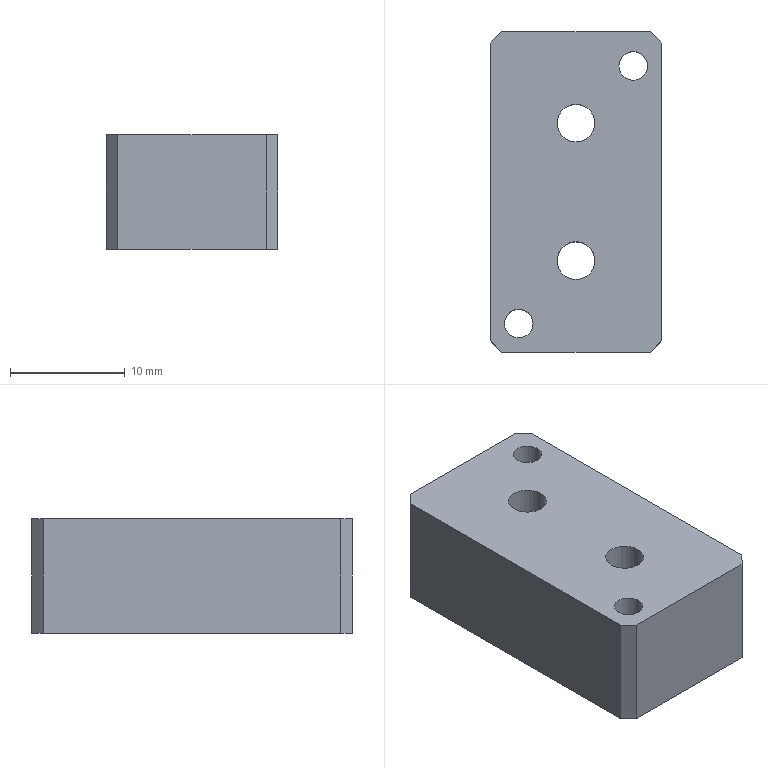Component | SolidWorks | JCT-03-04MicroSwitchMountingBlock-1 | 1 solid | 18 faces | box 15 x 28 x 10 mm | volume 3911 mm3 | plane 10 | cylinder 8 | commonest cylinder face diameters 2.5 x4 3.3 x4
build123d program:
from build123d import *

# Parameters (mm, degrees)
SKETCH1_W         = 15
SKETCH1_H         = 28
EXTRUDE1_DEPTH    = 5
M4_TAPPED_HOLE1_D = 3.3
M3_TAPPED_HOLE1_D = 2.5
CHAMFER1_SIZE     = 1


with BuildPart() as part:
    # Sketch1 → Extrude1 (new, symmetric)
    with BuildSketch(Plane.XY):
        Rectangle(SKETCH1_W, SKETCH1_H)
    extrude(amount=EXTRUDE1_DEPTH, both=True)

    # M4 Tapped Hole1 (through all)
    with Locations(Plane.XY.offset(5)):
        with Locations((0, -6), (0, 6)):
            Hole(M4_TAPPED_HOLE1_D / 2)

    # M3 Tapped Hole1 (through all)
    with Locations(Plane.XY.offset(5)):
        with Locations((5, 11), (-5, -11.5)):
            Hole(M3_TAPPED_HOLE1_D / 2)

    # Chamfer1
    chamfer1_edges = [part.edges().sort_by_distance(p)[0] for p in [
        (-7.5, 14, 0),
        (7.5, 14, 0),
        (7.5, -14, 0),
        (-7.5, -14, 0),
    ]]
    chamfer(chamfer1_edges, length=CHAMFER1_SIZE)


solid = part.part

# Placed as in the assembly
solid = solid.moved(Location((-12.734, 78.299, 51), (0, 0, 0)))
STEP:
#1=CARTESIAN_POINT('',(-0.3537,3.516,1.811));
#2=VERTEX_POINT('',#1);
#3=CARTESIAN_POINT('',(-0.2553,3.516,1.811));
#4=VERTEX_POINT('',#3);
#5=CARTESIAN_POINT('',(-0.3045,3.516,1.811));
#6=DIRECTION('',(0.,0.,1.));
#7=DIRECTION('',(1.,0.,0.));
#8=AXIS2_PLACEMENT_3D('',#5,#6,#7);
#9=CIRCLE('',#8,0.04921);
#10=EDGE_CURVE('',#2,#4,#9,.T.);
#11=ORIENTED_EDGE('',*,*,#10,.F.);
#12=CARTESIAN_POINT('',(-0.3537,3.516,2.205));
#13=VERTEX_POINT('',#12);
#14=CARTESIAN_POINT('',(-0.3537,3.516,2.205));
#15=DIRECTION('',(0.,0.,1.));
#16=VECTOR('',#15,39.37);
#17=LINE('',#14,#16);
#18=EDGE_CURVE('',#2,#13,#17,.T.);
#19=ORIENTED_EDGE('',*,*,#18,.T.);
#20=CARTESIAN_POINT('',(-0.2553,3.516,2.205));
#21=VERTEX_POINT('',#20);
#22=CARTESIAN_POINT('',(-0.3045,3.516,2.205));
#23=DIRECTION('',(0.,0.,1.));
#24=DIRECTION('',(1.,0.,0.));
#25=AXIS2_PLACEMENT_3D('',#22,#23,#24);
#26=CIRCLE('',#25,0.04921);
#27=EDGE_CURVE('',#13,#21,#26,.T.);
#28=ORIENTED_EDGE('',*,*,#27,.T.);
#29=CARTESIAN_POINT('',(-0.2553,3.516,2.205));
#30=DIRECTION('',(0.,0.,1.));
#31=VECTOR('',#30,39.37);
#32=LINE('',#29,#31);
#33=EDGE_CURVE('',#4,#21,#32,.T.);
#34=ORIENTED_EDGE('',*,*,#33,.F.);
#35=EDGE_LOOP('',(#11,#19,#28,#34));
#36=FACE_OUTER_BOUND('',#35,.T.);
#37=CARTESIAN_POINT('',(-0.3045,3.516,2.205));
#38=DIRECTION('',(0.,0.,1.));
#39=DIRECTION('',(1.,0.,0.));
#40=AXIS2_PLACEMENT_3D('',#37,#38,#39);
#41=CYLINDRICAL_SURFACE('',#40,0.04921);
#42=ADVANCED_FACE('',(#36),#41,.F.);
#43=CARTESIAN_POINT('',(-0.7474,2.63,1.811));
#44=VERTEX_POINT('',#43);
#45=CARTESIAN_POINT('',(-0.649,2.63,1.811));
#46=VERTEX_POINT('',#45);
#47=CARTESIAN_POINT('',(-0.6982,2.63,1.811));
#48=DIRECTION('',(0.,0.,1.));
#49=DIRECTION('',(1.,0.,0.));
#50=AXIS2_PLACEMENT_3D('',#47,#48,#49);
#51=CIRCLE('',#50,0.04921);
#52=EDGE_CURVE('',#44,#46,#51,.T.);
#53=ORIENTED_EDGE('',*,*,#52,.F.);
#54=CARTESIAN_POINT('',(-0.7474,2.63,2.205));
#55=VERTEX_POINT('',#54);
#56=CARTESIAN_POINT('',(-0.7474,2.63,2.205));
#57=DIRECTION('',(0.,0.,1.));
#58=VECTOR('',#57,39.37);
#59=LINE('',#56,#58);
#60=EDGE_CURVE('',#44,#55,#59,.T.);
#61=ORIENTED_EDGE('',*,*,#60,.T.);
#62=CARTESIAN_POINT('',(-0.649,2.63,2.205));
#63=VERTEX_POINT('',#62);
#64=CARTESIAN_POINT('',(-0.6982,2.63,2.205));
#65=DIRECTION('',(0.,0.,1.));
#66=DIRECTION('',(1.,0.,0.));
#67=AXIS2_PLACEMENT_3D('',#64,#65,#66);
#68=CIRCLE('',#67,0.04921);
#69=EDGE_CURVE('',#55,#63,#68,.T.);
#70=ORIENTED_EDGE('',*,*,#69,.T.);
#71=CARTESIAN_POINT('',(-0.649,2.63,2.205));
#72=DIRECTION('',(0.,0.,1.));
#73=VECTOR('',#72,39.37);
#74=LINE('',#71,#73);
#75=EDGE_CURVE('',#46,#63,#74,.T.);
#76=ORIENTED_EDGE('',*,*,#75,.F.);
#77=EDGE_LOOP('',(#53,#61,#70,#76));
#78=FACE_OUTER_BOUND('',#77,.T.);
#79=CARTESIAN_POINT('',(-0.6982,2.63,2.205));
#80=DIRECTION('',(0.,0.,1.));
#81=DIRECTION('',(1.,0.,0.));
#82=AXIS2_PLACEMENT_3D('',#79,#80,#81);
#83=CYLINDRICAL_SURFACE('',#82,0.04921);
#84=ADVANCED_FACE('',(#78),#83,.F.);
#85=CARTESIAN_POINT('',(-0.5663,3.319,1.811));
#86=VERTEX_POINT('',#85);
#87=CARTESIAN_POINT('',(-0.4364,3.319,1.811));
#88=VERTEX_POINT('',#87);
#89=CARTESIAN_POINT('',(-0.5013,3.319,1.811));
#90=DIRECTION('',(0.,0.,1.));
#91=DIRECTION('',(1.,0.,0.));
#92=AXIS2_PLACEMENT_3D('',#89,#90,#91);
#93=CIRCLE('',#92,0.06496);
#94=EDGE_CURVE('',#86,#88,#93,.T.);
#95=ORIENTED_EDGE('',*,*,#94,.F.);
#96=CARTESIAN_POINT('',(-0.5663,3.319,2.205));
#97=VERTEX_POINT('',#96);
#98=CARTESIAN_POINT('',(-0.5663,3.319,2.205));
#99=DIRECTION('',(0.,0.,1.));
#100=VECTOR('',#99,39.37);
#101=LINE('',#98,#100);
#102=EDGE_CURVE('',#86,#97,#101,.T.);
#103=ORIENTED_EDGE('',*,*,#102,.T.);
#104=CARTESIAN_POINT('',(-0.4364,3.319,2.205));
#105=VERTEX_POINT('',#104);
#106=CARTESIAN_POINT('',(-0.5013,3.319,2.205));
#107=DIRECTION('',(0.,0.,1.));
#108=DIRECTION('',(1.,0.,0.));
#109=AXIS2_PLACEMENT_3D('',#106,#107,#108);
#110=CIRCLE('',#109,0.06496);
#111=EDGE_CURVE('',#97,#105,#110,.T.);
#112=ORIENTED_EDGE('',*,*,#111,.T.);
#113=CARTESIAN_POINT('',(-0.4364,3.319,2.205));
#114=DIRECTION('',(0.,0.,1.));
#115=VECTOR('',#114,39.37);
#116=LINE('',#113,#115);
#117=EDGE_CURVE('',#88,#105,#116,.T.);
#118=ORIENTED_EDGE('',*,*,#117,.F.);
#119=EDGE_LOOP('',(#95,#103,#112,#118));
#120=FACE_OUTER_BOUND('',#119,.T.);
#121=CARTESIAN_POINT('',(-0.5013,3.319,2.205));
#122=DIRECTION('',(0.,0.,1.));
#123=DIRECTION('',(1.,0.,0.));
#124=AXIS2_PLACEMENT_3D('',#121,#122,#123);
#125=CYLINDRICAL_SURFACE('',#124,0.06496);
#126=ADVANCED_FACE('',(#120),#125,.F.);
#127=CARTESIAN_POINT('',(-0.5663,2.846,1.811));
#128=VERTEX_POINT('',#127);
#129=CARTESIAN_POINT('',(-0.4364,2.846,1.811));
#130=VERTEX_POINT('',#129);
#131=CARTESIAN_POINT('',(-0.5013,2.846,1.811));
#132=DIRECTION('',(0.,0.,1.));
#133=DIRECTION('',(1.,0.,0.));
#134=AXIS2_PLACEMENT_3D('',#131,#132,#133);
#135=CIRCLE('',#134,0.06496);
#136=EDGE_CURVE('',#128,#130,#135,.T.);
#137=ORIENTED_EDGE('',*,*,#136,.F.);
#138=CARTESIAN_POINT('',(-0.5663,2.846,2.205));
#139=VERTEX_POINT('',#138);
#140=CARTESIAN_POINT('',(-0.5663,2.846,2.205));
#141=DIRECTION('',(0.,0.,1.));
#142=VECTOR('',#141,39.37);
#143=LINE('',#140,#142);
#144=EDGE_CURVE('',#128,#139,#143,.T.);
#145=ORIENTED_EDGE('',*,*,#144,.T.);
#146=CARTESIAN_POINT('',(-0.4364,2.846,2.205));
#147=VERTEX_POINT('',#146);
#148=CARTESIAN_POINT('',(-0.5013,2.846,2.205));
#149=DIRECTION('',(0.,0.,1.));
#150=DIRECTION('',(1.,0.,0.));
#151=AXIS2_PLACEMENT_3D('',#148,#149,#150);
#152=CIRCLE('',#151,0.06496);
#153=EDGE_CURVE('',#139,#147,#152,.T.);
#154=ORIENTED_EDGE('',*,*,#153,.T.);
#155=CARTESIAN_POINT('',(-0.4364,2.846,2.205));
#156=DIRECTION('',(0.,0.,1.));
#157=VECTOR('',#156,39.37);
#158=LINE('',#155,#157);
#159=EDGE_CURVE('',#130,#147,#158,.T.);
#160=ORIENTED_EDGE('',*,*,#159,.F.);
#161=EDGE_LOOP('',(#137,#145,#154,#160));
#162=FACE_OUTER_BOUND('',#161,.T.);
#163=CARTESIAN_POINT('',(-0.5013,2.846,2.205));
#164=DIRECTION('',(0.,0.,1.));
#165=DIRECTION('',(1.,0.,0.));
#166=AXIS2_PLACEMENT_3D('',#163,#164,#165);
#167=CYLINDRICAL_SURFACE('',#166,0.06496);
#168=ADVANCED_FACE('',(#162),#167,.F.);
#169=CARTESIAN_POINT('',(-0.7966,3.594,1.811));
#170=VERTEX_POINT('',#169);
#171=CARTESIAN_POINT('',(-0.7966,2.571,1.811));
#172=VERTEX_POINT('',#171);
#173=CARTESIAN_POINT('',(-0.7966,3.634,1.811));
#174=DIRECTION('',(0.,-1.,0.));
#175=VECTOR('',#174,39.37);
#176=LINE('',#173,#175);
#177=EDGE_CURVE('',#170,#172,#176,.T.);
#178=ORIENTED_EDGE('',*,*,#177,.T.);
#179=CARTESIAN_POINT('',(-0.7966,2.571,2.205));
#180=VERTEX_POINT('',#179);
#181=CARTESIAN_POINT('',(-0.7966,2.571,2.205));
#182=DIRECTION('',(0.,0.,1.));
#183=VECTOR('',#182,39.37);
#184=LINE('',#181,#183);
#185=EDGE_CURVE('',#172,#180,#184,.T.);
#186=ORIENTED_EDGE('',*,*,#185,.T.);
#187=CARTESIAN_POINT('',(-0.7966,3.594,2.205));
#188=VERTEX_POINT('',#187);
#189=CARTESIAN_POINT('',(-0.7966,3.634,2.205));
#190=DIRECTION('',(0.,-1.,0.));
#191=VECTOR('',#190,39.37);
#192=LINE('',#189,#191);
#193=EDGE_CURVE('',#188,#180,#192,.T.);
#194=ORIENTED_EDGE('',*,*,#193,.F.);
#195=CARTESIAN_POINT('',(-0.7966,3.594,2.205));
#196=DIRECTION('',(0.,0.,-1.));
#197=VECTOR('',#196,39.37);
#198=LINE('',#195,#197);
#199=EDGE_CURVE('',#188,#170,#198,.T.);
#200=ORIENTED_EDGE('',*,*,#199,.T.);
#201=EDGE_LOOP('',(#178,#186,#194,#200));
#202=FACE_OUTER_BOUND('',#201,.T.);
#203=CARTESIAN_POINT('',(-0.7966,3.634,2.205));
#204=DIRECTION('',(1.,0.,0.));
#205=DIRECTION('',(0.,0.,-1.));
#206=AXIS2_PLACEMENT_3D('',#203,#204,#205);
#207=PLANE('',#206);
#208=ADVANCED_FACE('',(#202),#207,.F.);
#209=CARTESIAN_POINT('',(-0.7572,2.531,2.205));
#210=VERTEX_POINT('',#209);
#211=CARTESIAN_POINT('',(-0.2454,2.531,2.205));
#212=VERTEX_POINT('',#211);
#213=CARTESIAN_POINT('',(-0.7966,2.531,2.205));
#214=DIRECTION('',(1.,-0.,0.));
#215=VECTOR('',#214,39.37);
#216=LINE('',#213,#215);
#217=EDGE_CURVE('',#210,#212,#216,.T.);
#218=ORIENTED_EDGE('',*,*,#217,.F.);
#219=CARTESIAN_POINT('',(-0.7572,2.531,1.811));
#220=VERTEX_POINT('',#219);
#221=CARTESIAN_POINT('',(-0.7572,2.531,2.205));
#222=DIRECTION('',(0.,0.,-1.));
#223=VECTOR('',#222,39.37);
#224=LINE('',#221,#223);
#225=EDGE_CURVE('',#210,#220,#224,.T.);
#226=ORIENTED_EDGE('',*,*,#225,.T.);
#227=CARTESIAN_POINT('',(-0.2454,2.531,1.811));
#228=VERTEX_POINT('',#227);
#229=CARTESIAN_POINT('',(-0.7966,2.531,1.811));
#230=DIRECTION('',(1.,-0.,0.));
#231=VECTOR('',#230,39.37);
#232=LINE('',#229,#231);
#233=EDGE_CURVE('',#220,#228,#232,.T.);
#234=ORIENTED_EDGE('',*,*,#233,.T.);
#235=CARTESIAN_POINT('',(-0.2454,2.531,2.205));
#236=DIRECTION('',(0.,0.,1.));
#237=VECTOR('',#236,39.37);
#238=LINE('',#235,#237);
#239=EDGE_CURVE('',#228,#212,#238,.T.);
#240=ORIENTED_EDGE('',*,*,#239,.T.);
#241=EDGE_LOOP('',(#218,#226,#234,#240));
#242=FACE_OUTER_BOUND('',#241,.T.);
#243=CARTESIAN_POINT('',(-0.7966,2.531,2.205));
#244=DIRECTION('',(0.,1.,0.));
#245=DIRECTION('',(-1.,0.,0.));
#246=AXIS2_PLACEMENT_3D('',#243,#244,#245);
#247=PLANE('',#246);
#248=ADVANCED_FACE('',(#242),#247,.F.);
#249=CARTESIAN_POINT('',(-0.2061,2.571,2.205));
#250=VERTEX_POINT('',#249);
#251=CARTESIAN_POINT('',(-0.2061,3.594,2.205));
#252=VERTEX_POINT('',#251);
#253=CARTESIAN_POINT('',(-0.2061,3.634,2.205));
#254=DIRECTION('',(0.,1.,0.));
#255=VECTOR('',#254,39.37);
#256=LINE('',#253,#255);
#257=EDGE_CURVE('',#250,#252,#256,.T.);
#258=ORIENTED_EDGE('',*,*,#257,.F.);
#259=CARTESIAN_POINT('',(-0.2061,2.571,1.811));
#260=VERTEX_POINT('',#259);
#261=CARTESIAN_POINT('',(-0.2061,2.571,2.205));
#262=DIRECTION('',(0.,0.,-1.));
#263=VECTOR('',#262,39.37);
#264=LINE('',#261,#263);
#265=EDGE_CURVE('',#250,#260,#264,.T.);
#266=ORIENTED_EDGE('',*,*,#265,.T.);
#267=CARTESIAN_POINT('',(-0.2061,3.594,1.811));
#268=VERTEX_POINT('',#267);
#269=CARTESIAN_POINT('',(-0.2061,3.634,1.811));
#270=DIRECTION('',(0.,1.,0.));
#271=VECTOR('',#270,39.37);
#272=LINE('',#269,#271);
#273=EDGE_CURVE('',#260,#268,#272,.T.);
#274=ORIENTED_EDGE('',*,*,#273,.T.);
#275=CARTESIAN_POINT('',(-0.2061,3.594,2.205));
#276=DIRECTION('',(0.,0.,1.));
#277=VECTOR('',#276,39.37);
#278=LINE('',#275,#277);
#279=EDGE_CURVE('',#268,#252,#278,.T.);
#280=ORIENTED_EDGE('',*,*,#279,.T.);
#281=EDGE_LOOP('',(#258,#266,#274,#280));
#282=FACE_OUTER_BOUND('',#281,.T.);
#283=CARTESIAN_POINT('',(-0.2061,3.634,2.205));
#284=DIRECTION('',(-1.,0.,0.));
#285=DIRECTION('',(0.,0.,1.));
#286=AXIS2_PLACEMENT_3D('',#283,#284,#285);
#287=PLANE('',#286);
#288=ADVANCED_FACE('',(#282),#287,.F.);
#289=CARTESIAN_POINT('',(-0.2454,3.634,2.205));
#290=VERTEX_POINT('',#289);
#291=CARTESIAN_POINT('',(-0.7572,3.634,2.205));
#292=VERTEX_POINT('',#291);
#293=CARTESIAN_POINT('',(-0.7966,3.634,2.205));
#294=DIRECTION('',(-1.,0.,0.));
#295=VECTOR('',#294,39.37);
#296=LINE('',#293,#295);
#297=EDGE_CURVE('',#290,#292,#296,.T.);
#298=ORIENTED_EDGE('',*,*,#297,.F.);
#299=CARTESIAN_POINT('',(-0.2454,3.634,1.811));
#300=VERTEX_POINT('',#299);
#301=CARTESIAN_POINT('',(-0.2454,3.634,2.205));
#302=DIRECTION('',(0.,0.,-1.));
#303=VECTOR('',#302,39.37);
#304=LINE('',#301,#303);
#305=EDGE_CURVE('',#290,#300,#304,.T.);
#306=ORIENTED_EDGE('',*,*,#305,.T.);
#307=CARTESIAN_POINT('',(-0.7572,3.634,1.811));
#308=VERTEX_POINT('',#307);
#309=CARTESIAN_POINT('',(-0.7966,3.634,1.811));
#310=DIRECTION('',(-1.,0.,0.));
#311=VECTOR('',#310,39.37);
#312=LINE('',#309,#311);
#313=EDGE_CURVE('',#300,#308,#312,.T.);
#314=ORIENTED_EDGE('',*,*,#313,.T.);
#315=CARTESIAN_POINT('',(-0.7572,3.634,2.205));
#316=DIRECTION('',(0.,0.,1.));
#317=VECTOR('',#316,39.37);
#318=LINE('',#315,#317);
#319=EDGE_CURVE('',#308,#292,#318,.T.);
#320=ORIENTED_EDGE('',*,*,#319,.T.);
#321=EDGE_LOOP('',(#298,#306,#314,#320));
#322=FACE_OUTER_BOUND('',#321,.T.);
#323=CARTESIAN_POINT('',(-0.7966,3.634,2.205));
#324=DIRECTION('',(0.,-1.,0.));
#325=DIRECTION('',(0.,0.,-1.));
#326=AXIS2_PLACEMENT_3D('',#323,#324,#325);
#327=PLANE('',#326);
#328=ADVANCED_FACE('',(#322),#327,.F.);
#329=CARTESIAN_POINT('',(-0.3045,3.516,2.205));
#330=DIRECTION('',(0.,0.,1.));
#331=DIRECTION('',(1.,0.,0.));
#332=AXIS2_PLACEMENT_3D('',#329,#330,#331);
#333=CIRCLE('',#332,0.04921);
#334=EDGE_CURVE('',#21,#13,#333,.T.);
#335=ORIENTED_EDGE('',*,*,#334,.F.);
#336=ORIENTED_EDGE('',*,*,#27,.F.);
#337=EDGE_LOOP('',(#335,#336));
#338=FACE_BOUND('',#337,.T.);
#339=CARTESIAN_POINT('',(-0.6982,2.63,2.205));
#340=DIRECTION('',(0.,0.,1.));
#341=DIRECTION('',(1.,0.,0.));
#342=AXIS2_PLACEMENT_3D('',#339,#340,#341);
#343=CIRCLE('',#342,0.04921);
#344=EDGE_CURVE('',#63,#55,#343,.T.);
#345=ORIENTED_EDGE('',*,*,#344,.F.);
#346=ORIENTED_EDGE('',*,*,#69,.F.);
#347=EDGE_LOOP('',(#345,#346));
#348=FACE_BOUND('',#347,.T.);
#349=CARTESIAN_POINT('',(-0.5013,3.319,2.205));
#350=DIRECTION('',(0.,0.,1.));
#351=DIRECTION('',(1.,0.,0.));
#352=AXIS2_PLACEMENT_3D('',#349,#350,#351);
#353=CIRCLE('',#352,0.06496);
#354=EDGE_CURVE('',#105,#97,#353,.T.);
#355=ORIENTED_EDGE('',*,*,#354,.F.);
#356=ORIENTED_EDGE('',*,*,#111,.F.);
#357=EDGE_LOOP('',(#355,#356));
#358=FACE_BOUND('',#357,.T.);
#359=CARTESIAN_POINT('',(-0.5013,2.846,2.205));
#360=DIRECTION('',(0.,0.,1.));
#361=DIRECTION('',(1.,0.,0.));
#362=AXIS2_PLACEMENT_3D('',#359,#360,#361);
#363=CIRCLE('',#362,0.06496);
#364=EDGE_CURVE('',#147,#139,#363,.T.);
#365=ORIENTED_EDGE('',*,*,#364,.F.);
#366=ORIENTED_EDGE('',*,*,#153,.F.);
#367=EDGE_LOOP('',(#365,#366));
#368=FACE_BOUND('',#367,.T.);
#369=ORIENTED_EDGE('',*,*,#193,.T.);
#370=CARTESIAN_POINT('',(-0.7769,2.551,2.205));
#371=DIRECTION('',(0.7071,-0.7071,0.));
#372=VECTOR('',#371,39.37);
#373=LINE('',#370,#372);
#374=EDGE_CURVE('',#180,#210,#373,.T.);
#375=ORIENTED_EDGE('',*,*,#374,.T.);
#376=ORIENTED_EDGE('',*,*,#217,.T.);
#377=CARTESIAN_POINT('',(-0.521,2.256,2.205));
#378=DIRECTION('',(0.7071,0.7071,0.));
#379=VECTOR('',#378,39.37);
#380=LINE('',#377,#379);
#381=EDGE_CURVE('',#212,#250,#380,.T.);
#382=ORIENTED_EDGE('',*,*,#381,.T.);
#383=ORIENTED_EDGE('',*,*,#257,.T.);
#384=CARTESIAN_POINT('',(0.03017,3.358,2.205));
#385=DIRECTION('',(-0.7071,0.7071,0.));
#386=VECTOR('',#385,39.37);
#387=LINE('',#384,#386);
#388=EDGE_CURVE('',#252,#290,#387,.T.);
#389=ORIENTED_EDGE('',*,*,#388,.T.);
#390=ORIENTED_EDGE('',*,*,#297,.T.);
#391=CARTESIAN_POINT('',(-1.328,3.063,2.205));
#392=DIRECTION('',(-0.7071,-0.7071,0.));
#393=VECTOR('',#392,39.37);
#394=LINE('',#391,#393);
#395=EDGE_CURVE('',#292,#188,#394,.T.);
#396=ORIENTED_EDGE('',*,*,#395,.T.);
#397=EDGE_LOOP('',(#369,#375,#376,#382,#383,#389,#390,#396));
#398=FACE_OUTER_BOUND('',#397,.T.);
#399=CARTESIAN_POINT('',(-0.7966,2.531,2.205));
#400=DIRECTION('',(0.,0.,1.));
#401=DIRECTION('',(1.,0.,0.));
#402=AXIS2_PLACEMENT_3D('',#399,#400,#401);
#403=PLANE('',#402);
#404=ADVANCED_FACE('',(#338,#348,#358,#368,#398),#403,.T.);
#405=CARTESIAN_POINT('',(-0.3045,3.516,1.811));
#406=DIRECTION('',(0.,0.,1.));
#407=DIRECTION('',(1.,0.,0.));
#408=AXIS2_PLACEMENT_3D('',#405,#406,#407);
#409=CIRCLE('',#408,0.04921);
#410=EDGE_CURVE('',#4,#2,#409,.T.);
#411=ORIENTED_EDGE('',*,*,#410,.T.);
#412=ORIENTED_EDGE('',*,*,#10,.T.);
#413=EDGE_LOOP('',(#411,#412));
#414=FACE_BOUND('',#413,.T.);
#415=CARTESIAN_POINT('',(-0.6982,2.63,1.811));
#416=DIRECTION('',(0.,0.,1.));
#417=DIRECTION('',(1.,0.,0.));
#418=AXIS2_PLACEMENT_3D('',#415,#416,#417);
#419=CIRCLE('',#418,0.04921);
#420=EDGE_CURVE('',#46,#44,#419,.T.);
#421=ORIENTED_EDGE('',*,*,#420,.T.);
#422=ORIENTED_EDGE('',*,*,#52,.T.);
#423=EDGE_LOOP('',(#421,#422));
#424=FACE_BOUND('',#423,.T.);
#425=CARTESIAN_POINT('',(-0.5013,3.319,1.811));
#426=DIRECTION('',(0.,0.,1.));
#427=DIRECTION('',(1.,0.,0.));
#428=AXIS2_PLACEMENT_3D('',#425,#426,#427);
#429=CIRCLE('',#428,0.06496);
#430=EDGE_CURVE('',#88,#86,#429,.T.);
#431=ORIENTED_EDGE('',*,*,#430,.T.);
#432=ORIENTED_EDGE('',*,*,#94,.T.);
#433=EDGE_LOOP('',(#431,#432));
#434=FACE_BOUND('',#433,.T.);
#435=CARTESIAN_POINT('',(-0.5013,2.846,1.811));
#436=DIRECTION('',(0.,0.,1.));
#437=DIRECTION('',(1.,0.,0.));
#438=AXIS2_PLACEMENT_3D('',#435,#436,#437);
#439=CIRCLE('',#438,0.06496);
#440=EDGE_CURVE('',#130,#128,#439,.T.);
#441=ORIENTED_EDGE('',*,*,#440,.T.);
#442=ORIENTED_EDGE('',*,*,#136,.T.);
#443=EDGE_LOOP('',(#441,#442));
#444=FACE_BOUND('',#443,.T.);
#445=ORIENTED_EDGE('',*,*,#233,.F.);
#446=CARTESIAN_POINT('',(-0.7572,2.531,1.811));
#447=DIRECTION('',(-0.7071,0.7071,0.));
#448=VECTOR('',#447,39.37);
#449=LINE('',#446,#448);
#450=EDGE_CURVE('',#220,#172,#449,.T.);
#451=ORIENTED_EDGE('',*,*,#450,.T.);
#452=ORIENTED_EDGE('',*,*,#177,.F.);
#453=CARTESIAN_POINT('',(-0.7966,3.594,1.811));
#454=DIRECTION('',(0.7071,0.7071,0.));
#455=VECTOR('',#454,39.37);
#456=LINE('',#453,#455);
#457=EDGE_CURVE('',#170,#308,#456,.T.);
#458=ORIENTED_EDGE('',*,*,#457,.T.);
#459=ORIENTED_EDGE('',*,*,#313,.F.);
#460=CARTESIAN_POINT('',(-0.2454,3.634,1.811));
#461=DIRECTION('',(0.7071,-0.7071,0.));
#462=VECTOR('',#461,39.37);
#463=LINE('',#460,#462);
#464=EDGE_CURVE('',#300,#268,#463,.T.);
#465=ORIENTED_EDGE('',*,*,#464,.T.);
#466=ORIENTED_EDGE('',*,*,#273,.F.);
#467=CARTESIAN_POINT('',(-0.2061,2.571,1.811));
#468=DIRECTION('',(-0.7071,-0.7071,0.));
#469=VECTOR('',#468,39.37);
#470=LINE('',#467,#469);
#471=EDGE_CURVE('',#260,#228,#470,.T.);
#472=ORIENTED_EDGE('',*,*,#471,.T.);
#473=EDGE_LOOP('',(#445,#451,#452,#458,#459,#465,#466,#472));
#474=FACE_OUTER_BOUND('',#473,.T.);
#475=CARTESIAN_POINT('',(-0.7966,2.531,1.811));
#476=DIRECTION('',(0.,0.,1.));
#477=DIRECTION('',(1.,0.,0.));
#478=AXIS2_PLACEMENT_3D('',#475,#476,#477);
#479=PLANE('',#478);
#480=ADVANCED_FACE('',(#414,#424,#434,#444,#474),#479,.F.);
#481=ORIENTED_EDGE('',*,*,#144,.F.);
#482=ORIENTED_EDGE('',*,*,#440,.F.);
#483=ORIENTED_EDGE('',*,*,#159,.T.);
#484=ORIENTED_EDGE('',*,*,#364,.T.);
#485=EDGE_LOOP('',(#481,#482,#483,#484));
#486=FACE_OUTER_BOUND('',#485,.T.);
#487=CARTESIAN_POINT('',(-0.5013,2.846,2.205));
#488=DIRECTION('',(0.,0.,1.));
#489=DIRECTION('',(1.,0.,0.));
#490=AXIS2_PLACEMENT_3D('',#487,#488,#489);
#491=CYLINDRICAL_SURFACE('',#490,0.06496);
#492=ADVANCED_FACE('',(#486),#491,.F.);
#493=ORIENTED_EDGE('',*,*,#102,.F.);
#494=ORIENTED_EDGE('',*,*,#430,.F.);
#495=ORIENTED_EDGE('',*,*,#117,.T.);
#496=ORIENTED_EDGE('',*,*,#354,.T.);
#497=EDGE_LOOP('',(#493,#494,#495,#496));
#498=FACE_OUTER_BOUND('',#497,.T.);
#499=CARTESIAN_POINT('',(-0.5013,3.319,2.205));
#500=DIRECTION('',(0.,0.,1.));
#501=DIRECTION('',(1.,0.,0.));
#502=AXIS2_PLACEMENT_3D('',#499,#500,#501);
#503=CYLINDRICAL_SURFACE('',#502,0.06496);
#504=ADVANCED_FACE('',(#498),#503,.F.);
#505=ORIENTED_EDGE('',*,*,#60,.F.);
#506=ORIENTED_EDGE('',*,*,#420,.F.);
#507=ORIENTED_EDGE('',*,*,#75,.T.);
#508=ORIENTED_EDGE('',*,*,#344,.T.);
#509=EDGE_LOOP('',(#505,#506,#507,#508));
#510=FACE_OUTER_BOUND('',#509,.T.);
#511=CARTESIAN_POINT('',(-0.6982,2.63,2.205));
#512=DIRECTION('',(0.,0.,1.));
#513=DIRECTION('',(1.,0.,0.));
#514=AXIS2_PLACEMENT_3D('',#511,#512,#513);
#515=CYLINDRICAL_SURFACE('',#514,0.04921);
#516=ADVANCED_FACE('',(#510),#515,.F.);
#517=ORIENTED_EDGE('',*,*,#18,.F.);
#518=ORIENTED_EDGE('',*,*,#410,.F.);
#519=ORIENTED_EDGE('',*,*,#33,.T.);
#520=ORIENTED_EDGE('',*,*,#334,.T.);
#521=EDGE_LOOP('',(#517,#518,#519,#520));
#522=FACE_OUTER_BOUND('',#521,.T.);
#523=CARTESIAN_POINT('',(-0.3045,3.516,2.205));
#524=DIRECTION('',(0.,0.,1.));
#525=DIRECTION('',(1.,0.,0.));
#526=AXIS2_PLACEMENT_3D('',#523,#524,#525);
#527=CYLINDRICAL_SURFACE('',#526,0.04921);
#528=ADVANCED_FACE('',(#522),#527,.F.);
#529=ORIENTED_EDGE('',*,*,#374,.F.);
#530=ORIENTED_EDGE('',*,*,#185,.F.);
#531=ORIENTED_EDGE('',*,*,#450,.F.);
#532=ORIENTED_EDGE('',*,*,#225,.F.);
#533=EDGE_LOOP('',(#529,#530,#531,#532));
#534=FACE_OUTER_BOUND('',#533,.T.);
#535=CARTESIAN_POINT('',(-0.7572,2.531,2.205));
#536=DIRECTION('',(0.7071,0.7071,0.));
#537=DIRECTION('',(-0.7071,0.7071,0.));
#538=AXIS2_PLACEMENT_3D('',#535,#536,#537);
#539=PLANE('',#538);
#540=ADVANCED_FACE('',(#534),#539,.F.);
#541=ORIENTED_EDGE('',*,*,#381,.F.);
#542=ORIENTED_EDGE('',*,*,#239,.F.);
#543=ORIENTED_EDGE('',*,*,#471,.F.);
#544=ORIENTED_EDGE('',*,*,#265,.F.);
#545=EDGE_LOOP('',(#541,#542,#543,#544));
#546=FACE_OUTER_BOUND('',#545,.T.);
#547=CARTESIAN_POINT('',(-0.2061,2.571,2.205));
#548=DIRECTION('',(-0.7071,0.7071,0.));
#549=DIRECTION('',(-0.7071,-0.7071,0.));
#550=AXIS2_PLACEMENT_3D('',#547,#548,#549);
#551=PLANE('',#550);
#552=ADVANCED_FACE('',(#546),#551,.F.);
#553=ORIENTED_EDGE('',*,*,#388,.F.);
#554=ORIENTED_EDGE('',*,*,#279,.F.);
#555=ORIENTED_EDGE('',*,*,#464,.F.);
#556=ORIENTED_EDGE('',*,*,#305,.F.);
#557=EDGE_LOOP('',(#553,#554,#555,#556));
#558=FACE_OUTER_BOUND('',#557,.T.);
#559=CARTESIAN_POINT('',(-0.2454,3.634,2.205));
#560=DIRECTION('',(-0.7071,-0.7071,0.));
#561=DIRECTION('',(0.7071,-0.7071,0.));
#562=AXIS2_PLACEMENT_3D('',#559,#560,#561);
#563=PLANE('',#562);
#564=ADVANCED_FACE('',(#558),#563,.F.);
#565=ORIENTED_EDGE('',*,*,#395,.F.);
#566=ORIENTED_EDGE('',*,*,#319,.F.);
#567=ORIENTED_EDGE('',*,*,#457,.F.);
#568=ORIENTED_EDGE('',*,*,#199,.F.);
#569=EDGE_LOOP('',(#565,#566,#567,#568));
#570=FACE_OUTER_BOUND('',#569,.T.);
#571=CARTESIAN_POINT('',(-0.7966,3.594,2.205));
#572=DIRECTION('',(0.7071,-0.7071,0.));
#573=DIRECTION('',(0.7071,0.7071,0.));
#574=AXIS2_PLACEMENT_3D('',#571,#572,#573);
#575=PLANE('',#574);
#576=ADVANCED_FACE('',(#570),#575,.F.);
#577=CLOSED_SHELL('',(#42,#84,#126,#168,#208,#248,#288,#328,#404,#480,#492,#504,#516,#528,#540,#552,#564,#576));
#578=MANIFOLD_SOLID_BREP('',#577);
#579=CARTESIAN_POINT('',(0.,0.,0.));
#580=DIRECTION('',(0.,0.,1.));
#581=DIRECTION('',(1.,0.,0.));
#582=AXIS2_PLACEMENT_3D('',#579,#580,#581);
#583=(LENGTH_UNIT()NAMED_UNIT(*)SI_UNIT($,.METRE.));
#584=LENGTH_MEASURE_WITH_UNIT(LENGTH_MEASURE(0.0254),#583);
#585=DIMENSIONAL_EXPONENTS(1.,0.,0.,0.,0.,0.,0.);
#586=(CONVERSION_BASED_UNIT('',#584)LENGTH_UNIT()NAMED_UNIT(#585));
#587=UNCERTAINTY_MEASURE_WITH_UNIT(LENGTH_MEASURE(0.00001),#586,'','');
#588=(NAMED_UNIT(*)PLANE_ANGLE_UNIT()SI_UNIT($,.RADIAN.));
#589=(NAMED_UNIT(*)SI_UNIT($,.STERADIAN.)SOLID_ANGLE_UNIT());
#590=(GEOMETRIC_REPRESENTATION_CONTEXT(3)GLOBAL_UNCERTAINTY_ASSIGNED_CONTEXT((#587))GLOBAL_UNIT_ASSIGNED_CONTEXT((#586,#588,#589))REPRESENTATION_CONTEXT('',''));
#591=ADVANCED_BREP_SHAPE_REPRESENTATION('',(#578,#582),#590);
#592=COLOUR_RGB('',0.7922,0.8196,0.9333);
#593=FILL_AREA_STYLE_COLOUR('',#592);
#594=FILL_AREA_STYLE('',(#593));
#595=SURFACE_STYLE_FILL_AREA(#594);
#596=SURFACE_SIDE_STYLE('',(#595));
#597=SURFACE_STYLE_USAGE(.BOTH.,#596);
#598=PRESENTATION_STYLE_ASSIGNMENT((#597));
#599=STYLED_ITEM('',(#598),#578);
#600=(LENGTH_UNIT()NAMED_UNIT(*)SI_UNIT($,.METRE.));
#601=LENGTH_MEASURE_WITH_UNIT(LENGTH_MEASURE(0.0254),#600);
#602=DIMENSIONAL_EXPONENTS(1.,0.,0.,0.,0.,0.,0.);
#603=(CONVERSION_BASED_UNIT('',#601)LENGTH_UNIT()NAMED_UNIT(#602));
#604=UNCERTAINTY_MEASURE_WITH_UNIT(LENGTH_MEASURE(0.00001),#603,'','');
#605=(NAMED_UNIT(*)PLANE_ANGLE_UNIT()SI_UNIT($,.RADIAN.));
#606=(NAMED_UNIT(*)SI_UNIT($,.STERADIAN.)SOLID_ANGLE_UNIT());
#607=(GEOMETRIC_REPRESENTATION_CONTEXT(3)GLOBAL_UNCERTAINTY_ASSIGNED_CONTEXT((#604))GLOBAL_UNIT_ASSIGNED_CONTEXT((#603,#605,#606))REPRESENTATION_CONTEXT('',''));
#608=MECHANICAL_DESIGN_GEOMETRIC_PRESENTATION_REPRESENTATION('',(#599),#607);
#609=PRESENTATION_LAYER_ASSIGNMENT('','',(#599));